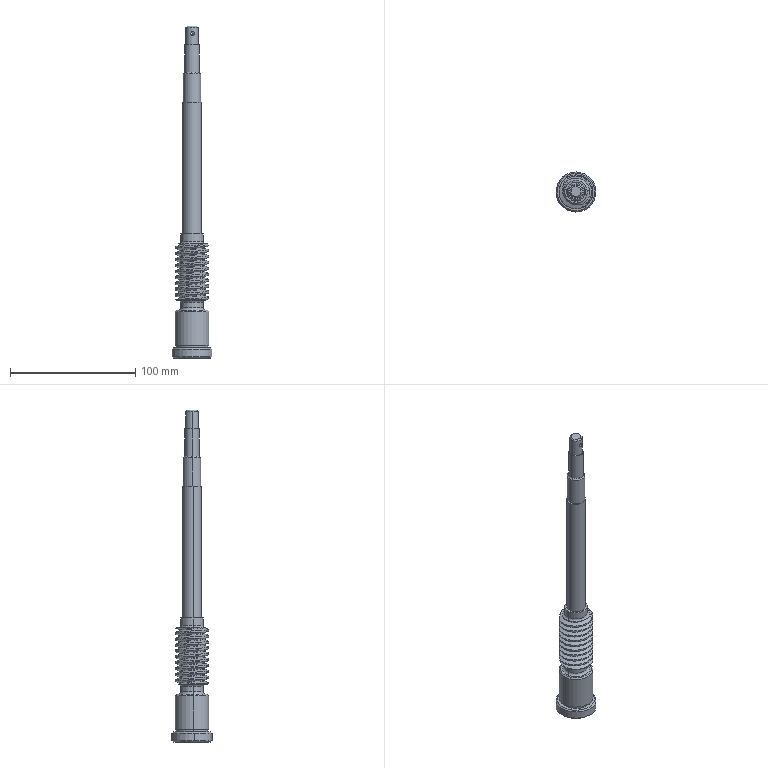Component | SolidWorks | 12Turbine-1 | 1 solid | 94 faces | volume 73453 mm3 | cylinder 59 | cone 16 | plane 11 | torus 6 | spline 2 | commonest cylinder face diameters 27 x22 20.25 x21 18 x4 10 x2 11.5 x2 14 x2 15 x2 25 x2